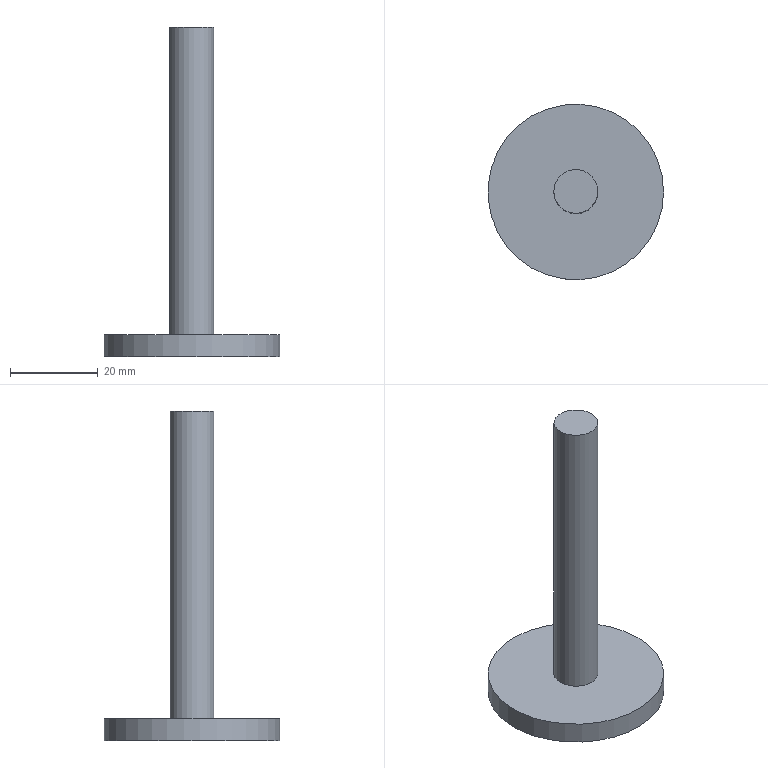Component | NX | PISTON_2 | 1 solid | 5 faces | box 40 x 40 x 75 mm | volume 11781 mm3 | plane 3 | cylinder 2 | commonest cylinder face diameters 40 x1 10 x1
STEP:
#1=CARTESIAN_POINT('',(0.,0.,0.));
#2=DIRECTION('',(0.,0.,1.));
#3=DIRECTION('',(1.,0.,0.));
#4=AXIS2_PLACEMENT_3D('',#1,#2,#3);
#5=CARTESIAN_POINT('',(-280.,0.,47.303));
#6=VERTEX_POINT('',#5);
#7=CARTESIAN_POINT('',(-285.,0.,47.303));
#8=DIRECTION('',(0.,0.,1.));
#9=DIRECTION('',(1.,0.,0.));
#10=AXIS2_PLACEMENT_3D('',#7,#8,#9);
#11=CIRCLE('',#10,5.);
#12=CARTESIAN_POINT('',(-285.,0.,47.303));
#13=DIRECTION('',(0.,0.,1.));
#14=DIRECTION('',(1.,0.,0.));
#15=AXIS2_PLACEMENT_3D('',#12,#13,#14);
#16=PLANE('',#15);
#17=CARTESIAN_POINT('',(0.,0.));
#18=DIRECTION('',(1.,0.));
#19=AXIS2_PLACEMENT_2D('',#17,#18);
#20=CIRCLE('',#19,5.);
#21=(GEOMETRIC_REPRESENTATION_CONTEXT(2)PARAMETRIC_REPRESENTATION_CONTEXT()REPRESENTATION_CONTEXT('',''));
#22=DEFINITIONAL_REPRESENTATION('',(#20),#21);
#23=PCURVE('',#16,#22);
#24=CARTESIAN_POINT('',(-285.,0.,42.303));
#25=DIRECTION('',(0.,0.,1.));
#26=DIRECTION('',(1.,0.,0.));
#27=AXIS2_PLACEMENT_3D('',#24,#25,#26);
#28=CYLINDRICAL_SURFACE('',#27,5.);
#29=CARTESIAN_POINT('',(0.,5.));
#30=DIRECTION('',(1.,0.));
#31=VECTOR('',#30,1.);
#32=LINE('',#29,#31);
#33=(GEOMETRIC_REPRESENTATION_CONTEXT(2)PARAMETRIC_REPRESENTATION_CONTEXT()REPRESENTATION_CONTEXT('',''));
#34=DEFINITIONAL_REPRESENTATION('',(#32),#33);
#35=PCURVE('',#28,#34);
#36=SURFACE_CURVE('',#11,(#23,#35),.PCURVE_S1.);
#37=EDGE_CURVE('',#6,#6,#36,.T.);
#38=ORIENTED_EDGE('',*,*,#37,.F.);
#39=EDGE_LOOP('',(#38));
#40=FACE_BOUND('',#39,.T.);
#41=CARTESIAN_POINT('',(-265.,0.,47.303));
#42=VERTEX_POINT('',#41);
#43=CARTESIAN_POINT('',(-285.,0.,47.303));
#44=DIRECTION('',(0.,0.,-1.));
#45=DIRECTION('',(1.,0.,0.));
#46=AXIS2_PLACEMENT_3D('',#43,#44,#45);
#47=CIRCLE('',#46,20.);
#48=CARTESIAN_POINT('',(20.,0.));
#49=CARTESIAN_POINT('',(20.,-34.641));
#50=CARTESIAN_POINT('',(-10.,-17.321));
#51=CARTESIAN_POINT('',(-40.,-0.));
#52=CARTESIAN_POINT('',(-10.,17.321));
#53=CARTESIAN_POINT('',(20.,34.641));
#54=CARTESIAN_POINT('',(20.,0.));
#55=(BOUNDED_CURVE()B_SPLINE_CURVE(2,(#48,#49,#50,#51,#52,#53,#54),.UNSPECIFIED.,.T.,.F.)B_SPLINE_CURVE_WITH_KNOTS((1,2,2,2,2,1),(-2.094,0.,2.094,4.189,6.283,8.378),.UNSPECIFIED.)CURVE()GEOMETRIC_REPRESENTATION_ITEM()RATIONAL_B_SPLINE_CURVE((1.,0.5,1.,0.5,1.,0.5,1.))REPRESENTATION_ITEM(''));
#56=(GEOMETRIC_REPRESENTATION_CONTEXT(2)PARAMETRIC_REPRESENTATION_CONTEXT()REPRESENTATION_CONTEXT('',''));
#57=DEFINITIONAL_REPRESENTATION('',(#55),#56);
#58=PCURVE('',#16,#57);
#59=CARTESIAN_POINT('',(-285.,0.,42.303));
#60=DIRECTION('',(0.,0.,1.));
#61=DIRECTION('',(1.,0.,0.));
#62=AXIS2_PLACEMENT_3D('',#59,#60,#61);
#63=CYLINDRICAL_SURFACE('',#62,20.);
#64=CARTESIAN_POINT('',(6.283,5.));
#65=DIRECTION('',(-1.,0.));
#66=VECTOR('',#65,1.);
#67=LINE('',#64,#66);
#68=(GEOMETRIC_REPRESENTATION_CONTEXT(2)PARAMETRIC_REPRESENTATION_CONTEXT()REPRESENTATION_CONTEXT('',''));
#69=DEFINITIONAL_REPRESENTATION('',(#67),#68);
#70=PCURVE('',#63,#69);
#71=SURFACE_CURVE('',#47,(#58,#70),.PCURVE_S1.);
#72=EDGE_CURVE('',#42,#42,#71,.T.);
#73=ORIENTED_EDGE('',*,*,#72,.F.);
#74=EDGE_LOOP('',(#73));
#75=FACE_BOUND('',#74,.T.);
#76=ADVANCED_FACE('',(#40,#75),#16,.T.);
#77=CARTESIAN_POINT('',(-265.,0.,42.303));
#78=VERTEX_POINT('',#77);
#79=CARTESIAN_POINT('',(-285.,0.,42.303));
#80=DIRECTION('',(0.,0.,1.));
#81=DIRECTION('',(1.,0.,0.));
#82=AXIS2_PLACEMENT_3D('',#79,#80,#81);
#83=CIRCLE('',#82,20.);
#84=CARTESIAN_POINT('',(-285.,0.,42.303));
#85=DIRECTION('',(0.,0.,-1.));
#86=DIRECTION('',(-1.,0.,0.));
#87=AXIS2_PLACEMENT_3D('',#84,#85,#86);
#88=PLANE('',#87);
#89=CARTESIAN_POINT('',(-20.,0.));
#90=CARTESIAN_POINT('',(-20.,34.641));
#91=CARTESIAN_POINT('',(10.,17.321));
#92=CARTESIAN_POINT('',(40.,0.));
#93=CARTESIAN_POINT('',(10.,-17.321));
#94=CARTESIAN_POINT('',(-20.,-34.641));
#95=CARTESIAN_POINT('',(-20.,0.));
#96=(BOUNDED_CURVE()B_SPLINE_CURVE(2,(#89,#90,#91,#92,#93,#94,#95),.UNSPECIFIED.,.T.,.F.)B_SPLINE_CURVE_WITH_KNOTS((1,2,2,2,2,1),(-2.094,0.,2.094,4.189,6.283,8.378),.UNSPECIFIED.)CURVE()GEOMETRIC_REPRESENTATION_ITEM()RATIONAL_B_SPLINE_CURVE((1.,0.5,1.,0.5,1.,0.5,1.))REPRESENTATION_ITEM(''));
#97=(GEOMETRIC_REPRESENTATION_CONTEXT(2)PARAMETRIC_REPRESENTATION_CONTEXT()REPRESENTATION_CONTEXT('',''));
#98=DEFINITIONAL_REPRESENTATION('',(#96),#97);
#99=PCURVE('',#88,#98);
#100=CARTESIAN_POINT('',(0.,0.));
#101=DIRECTION('',(1.,0.));
#102=VECTOR('',#101,1.);
#103=LINE('',#100,#102);
#104=(GEOMETRIC_REPRESENTATION_CONTEXT(2)PARAMETRIC_REPRESENTATION_CONTEXT()REPRESENTATION_CONTEXT('',''));
#105=DEFINITIONAL_REPRESENTATION('',(#103),#104);
#106=PCURVE('',#63,#105);
#107=SURFACE_CURVE('',#83,(#99,#106),.PCURVE_S1.);
#108=EDGE_CURVE('',#78,#78,#107,.T.);
#109=ORIENTED_EDGE('',*,*,#108,.F.);
#110=EDGE_LOOP('',(#109));
#111=FACE_BOUND('',#110,.T.);
#112=ADVANCED_FACE('',(#111),#88,.T.);
#113=ORIENTED_EDGE('',*,*,#72,.T.);
#114=CARTESIAN_POINT('',(-265.,0.,42.303));
#115=CARTESIAN_POINT('',(-265.,0.,47.303));
#116=B_SPLINE_CURVE_WITH_KNOTS('',1,(#114,#115),.UNSPECIFIED.,.F.,.F.,(2,2),(0.,5.),.PIECEWISE_BEZIER_KNOTS.);
#117=CARTESIAN_POINT('',(0.,0.));
#118=DIRECTION('',(0.,1.));
#119=VECTOR('',#118,1.);
#120=LINE('',#117,#119);
#121=(GEOMETRIC_REPRESENTATION_CONTEXT(2)PARAMETRIC_REPRESENTATION_CONTEXT()REPRESENTATION_CONTEXT('',''));
#122=DEFINITIONAL_REPRESENTATION('',(#120),#121);
#123=PCURVE('',#63,#122);
#124=CARTESIAN_POINT('',(6.283,0.));
#125=DIRECTION('',(0.,1.));
#126=VECTOR('',#125,1.);
#127=LINE('',#124,#126);
#128=(GEOMETRIC_REPRESENTATION_CONTEXT(2)PARAMETRIC_REPRESENTATION_CONTEXT()REPRESENTATION_CONTEXT('',''));
#129=DEFINITIONAL_REPRESENTATION('',(#127),#128);
#130=PCURVE('',#63,#129);
#131=SEAM_CURVE('',#116,(#123,#130),.PCURVE_S1.);
#132=EDGE_CURVE('',#78,#42,#131,.T.);
#133=ORIENTED_EDGE('',*,*,#132,.F.);
#134=ORIENTED_EDGE('',*,*,#108,.T.);
#135=ORIENTED_EDGE('',*,*,#132,.T.);
#136=EDGE_LOOP('',(#113,#133,#134,#135));
#137=FACE_BOUND('',#136,.T.);
#138=ADVANCED_FACE('',(#137),#63,.T.);
#139=CARTESIAN_POINT('',(-280.,0.,117.303));
#140=VERTEX_POINT('',#139);
#141=CARTESIAN_POINT('',(-285.,0.,117.303));
#142=DIRECTION('',(0.,0.,1.));
#143=DIRECTION('',(1.,0.,0.));
#144=AXIS2_PLACEMENT_3D('',#141,#142,#143);
#145=CIRCLE('',#144,5.);
#146=CARTESIAN_POINT('',(-285.,0.,117.303));
#147=DIRECTION('',(0.,0.,1.));
#148=DIRECTION('',(1.,0.,0.));
#149=AXIS2_PLACEMENT_3D('',#146,#147,#148);
#150=PLANE('',#149);
#151=CARTESIAN_POINT('',(0.,0.));
#152=DIRECTION('',(1.,0.));
#153=AXIS2_PLACEMENT_2D('',#151,#152);
#154=CIRCLE('',#153,5.);
#155=(GEOMETRIC_REPRESENTATION_CONTEXT(2)PARAMETRIC_REPRESENTATION_CONTEXT()REPRESENTATION_CONTEXT('',''));
#156=DEFINITIONAL_REPRESENTATION('',(#154),#155);
#157=PCURVE('',#150,#156);
#158=CARTESIAN_POINT('',(0.,75.));
#159=DIRECTION('',(1.,0.));
#160=VECTOR('',#159,1.);
#161=LINE('',#158,#160);
#162=(GEOMETRIC_REPRESENTATION_CONTEXT(2)PARAMETRIC_REPRESENTATION_CONTEXT()REPRESENTATION_CONTEXT('',''));
#163=DEFINITIONAL_REPRESENTATION('',(#161),#162);
#164=PCURVE('',#28,#163);
#165=SURFACE_CURVE('',#145,(#157,#164),.PCURVE_S1.);
#166=EDGE_CURVE('',#140,#140,#165,.T.);
#167=ORIENTED_EDGE('',*,*,#166,.T.);
#168=EDGE_LOOP('',(#167));
#169=FACE_BOUND('',#168,.T.);
#170=ADVANCED_FACE('',(#169),#150,.T.);
#171=ORIENTED_EDGE('',*,*,#37,.T.);
#172=CARTESIAN_POINT('',(-280.,0.,47.303));
#173=CARTESIAN_POINT('',(-280.,0.,117.303));
#174=B_SPLINE_CURVE_WITH_KNOTS('',1,(#172,#173),.UNSPECIFIED.,.F.,.F.,(2,2),(5.,75.),.PIECEWISE_BEZIER_KNOTS.);
#175=CARTESIAN_POINT('',(6.283,0.));
#176=DIRECTION('',(0.,1.));
#177=VECTOR('',#176,1.);
#178=LINE('',#175,#177);
#179=(GEOMETRIC_REPRESENTATION_CONTEXT(2)PARAMETRIC_REPRESENTATION_CONTEXT()REPRESENTATION_CONTEXT('',''));
#180=DEFINITIONAL_REPRESENTATION('',(#178),#179);
#181=PCURVE('',#28,#180);
#182=CARTESIAN_POINT('',(0.,0.));
#183=DIRECTION('',(0.,1.));
#184=VECTOR('',#183,1.);
#185=LINE('',#182,#184);
#186=(GEOMETRIC_REPRESENTATION_CONTEXT(2)PARAMETRIC_REPRESENTATION_CONTEXT()REPRESENTATION_CONTEXT('',''));
#187=DEFINITIONAL_REPRESENTATION('',(#185),#186);
#188=PCURVE('',#28,#187);
#189=SEAM_CURVE('',#174,(#181,#188),.PCURVE_S1.);
#190=EDGE_CURVE('',#6,#140,#189,.T.);
#191=ORIENTED_EDGE('',*,*,#190,.T.);
#192=ORIENTED_EDGE('',*,*,#166,.F.);
#193=ORIENTED_EDGE('',*,*,#190,.F.);
#194=EDGE_LOOP('',(#171,#191,#192,#193));
#195=FACE_BOUND('',#194,.T.);
#196=ADVANCED_FACE('',(#195),#28,.T.);
#197=CLOSED_SHELL('',(#76,#112,#138,#170,#196));
#198=MANIFOLD_SOLID_BREP('',#197);
#199=(LENGTH_UNIT()NAMED_UNIT(*)SI_UNIT(.MILLI.,.METRE.));
#200=UNCERTAINTY_MEASURE_WITH_UNIT(LENGTH_MEASURE(0.00001),#199,'','');
#201=(NAMED_UNIT(*)PLANE_ANGLE_UNIT()SI_UNIT($,.RADIAN.));
#202=(NAMED_UNIT(*)SI_UNIT($,.STERADIAN.)SOLID_ANGLE_UNIT());
#203=(GEOMETRIC_REPRESENTATION_CONTEXT(3)GLOBAL_UNCERTAINTY_ASSIGNED_CONTEXT((#200))GLOBAL_UNIT_ASSIGNED_CONTEXT((#199,#201,#202))REPRESENTATION_CONTEXT('',''));
#204=ADVANCED_BREP_SHAPE_REPRESENTATION('',(#4,#198),#203);